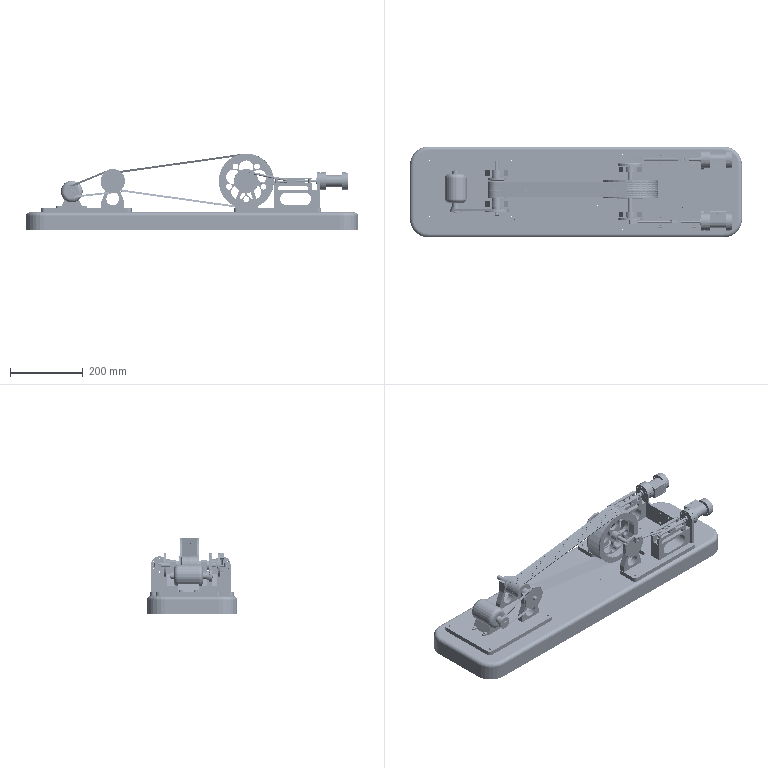Assembly | NX | mm | 63 component files | 63 solids | 1003 faces | box 915 x 250 x 212 mm | volume 14019484 mm3 | plane 402 | cylinder 384 | cone 186 | torus 16 | spline 15 | commonest cylinder face diameters 4 x86 3.3 x44 6 x42 5 x24 3 x24 12 x18 25 x18 10 x18
Bill of materials:
unnamed part 1 | 2 |  | Rectangular block with an obround (stadium-shaped) through-slot across its large side faces, four small holes on the top face near the ends, and two larger holes on one end face.
unnamed part 2 | 1 |  | Thin flat plate with rounded outer corners and a rectangular U-shaped notch with filleted inner corners cut into one edge; twelve small through-holes are spread across the plate.
unnamed part 3 | 2 |  | Rectangular flat plate with four through-holes, one near each corner.
unnamed part 4 | 4 |  | Thin circular ring (flat annulus) with a narrow rectangular-like cross-section.
unnamed part 5 | 1 |  | Single-groove V-profile pulley/sheave disc with a cylindrical hub protruding from one face and a central through-bore.
unnamed part 6 | 4 |  | Flat rectangular bar/strip with one through-hole near each end.
unnamed part 7 | 4 |  | Bridge-shaped bar with an inverted-U profile: a long top beam with a short leg at each end, filleted inner corners, and one vertical through-hole near each end on the top face.
unnamed part 8 | 2 |  | Circular disc with a central through-hole, a smaller off-center through-hole near the rim, and a shallow low boss on one face.
unnamed part 9 | 2 |  | Short solid cylinder with two rectangular circumferential grooves and a small central through-bore; one outer edge appears lightly chamfered.
unnamed part 10 | 1 |  | Thin flat plate with two raised rounded lobes at its ends; each lobe has a large central hole surrounded by six small holes, and the main body has eight medium holes in two rows. The inner corners between the lobes are filleted.
unnamed part 11 | 2 |  | Stepped cylindrical rod/shaft: a long main diameter with a short reduced-diameter section at one end.
unnamed part 12 | 1 |  | Cylindrical body with a bellows-like zigzag (convoluted) outer profile between two end flanges, plus a cylindrical hub at each end. It has a central through-bore and a small radial cross-hole in each hub.
unnamed part 13 | 1 |  | Long, slender solid cylindrical shaft or pin. Both ends step down to a short section of smaller diameter.
unnamed part 14 | 1 |  | Wheel shaped like a pulley. Its outer rim has several circumferential V-profile grooves. Inside the rim is a recessed web with five large and five small round lightening holes, around a central hub boss with a bore.
unnamed part 15 | 1 |  | Horizontal cylindrical body with rounded ends and a through-bore on its axis. It sits on a pedestal with tapered sides and a flat base. The base has four eared mounting tabs, each with a hole.
unnamed part 16 | 7 |  | Thin closed loop band with a teardrop shape. One end has a large rounded curve and the other a small rounded curve, joined by two straight tangent runs.
unnamed part 17 | 1 |  | Flat rectangular plate with rounded corners and twelve small through-holes. There is one hole near each corner. The other eight form two rectangular groups of four, each group with different spacing.
unnamed part 18 | 2 |  | Link made of a slender round rod joining two block-shaped end eyes. One block has a larger hole and chamfered corners. The other block has a rounded end and a smaller hole.
unnamed part 19 | 2 |  | Rectangular block with a rectangular notch cut in from one side, giving a U/C shape in plan. Round cross-holes pass through the side faces. A narrow rib or tongue projects from the bottom face.
unnamed part 20 | 1 |  | Stepped round shaft. One end has a collar and a short pilot spigot. The other end has stepped shoulders, a V-grooved sheave-like flange and a small end spigot.
unnamed part 21 | 2 |  | Housing with a rectangular box-shaped centre between two round end flanges. A large bore runs through along the axis. Each flange has six bolt holes in a circle. The box faces carry small holes and a set of short slots.
unnamed part 22 | 2 |  | Circular flange disc with a central bore and six bolt holes in a circle. A cylindrical hub projects from one face and a short raised face sits on the other.
unnamed part 23 | 8 |  | Plain cylindrical tube or bushing with a concentric through-bore and flat ends.
unnamed part 24 | 2 |  | Solid circular disc (blind-flange style) with six bolt holes in a circle and no central bore. A shallow raised face sits on one side and the edge is slightly chamfered.
unnamed part 25 | 4 |  | Flat plate of constant thickness with a bracket-like outline: a short semicircular lobe on top, a rectangular upper section, sides that flare outward lower down, and a rectangular base. It has a small round through-hole near the top and a large pear-shaped through-cutout below it, narrow at the top and wide and round at the bottom.
unnamed part 26 | 1 |  | Thin, long rectangular slab or pad with rounded corners in plan view and rounded or filleted edges around the top face. The bottom edge looks sharp.
unnamed part 27 | 1 |  | Long solid cylindrical rod with flat ends and two pairs of small cylindrical pins sticking out sideways. The pairs sit at two places along the rod, and in each pair the pins point in opposite directions.
unnamed part 28 | 1 |  | Thin closed-loop band with a uniform cross-section, shaped like a teardrop: a large rounded end and a small rounded end joined by two straight, converging sides. It is open in the middle and has no web.
Mates:
1. fix | base 1 component
2. concentric | base 1 arc | base_plate_1 1 edge
3. parallel | base_plate_1 1 face | base 1 face
4. concentric | support_block 2 edge | base_plate_1 1 edge
5. parallel | support_block 2 face | base_plate_1 1 face
6. parallel | support_block 1 face | support_block 2 face
7. concentric | support_block 1 edge | leg 4 edge
8. parallel | leg 4 face | support_block 1 face
9. concentric | support_block 1 edge | leg 3 edge
10. parallel | leg 3 face | support_block 1 face
11. concentric | support_block 2 edge | leg 2 edge
12. parallel | leg 2 face | support_block 2 face
13. concentric | support_block 2 edge | leg 1 edge
14. parallel | leg 1 face | support_block 2 face
15. concentric | fixed_post 8 arc | leg 4 edge
16. concentric | fixed_post 7 arc | leg 4 edge
17. concentric | fixed_post 6 arc | leg 3 edge
18. concentric | fixed_post 5 arc | leg 3 edge
19. concentric | fixed_post 8 edge | guide_plate 4 arc
20. parallel | guide_plate 4 face | leg 4 face
21. concentric | fixed_post 6 edge | guide_plate 3 arc
22. parallel | guide_plate 3 face | support_block 1 face
23. concentric | fixed_post 4 arc | leg 2 edge
24. concentric | fixed_post 3 arc | leg 2 edge
25. concentric | fixed_post 2 arc | leg 1 edge
26. concentric | fixed_post 1 arc | leg 1 edge
27. concentric | fixed_post 4 edge | guide_plate 2 arc
28. parallel | guide_plate 2 face | leg 2 face
29. concentric | fixed_post 2 edge | guide_plate 1 arc
30. parallel | guide_plate 1 face | leg 1 face
31. concentric | support_block 2 edge | piston_cylinder_mount_plate 1 arc
32. parallel | piston_cylinder_mount_plate 1 face | base 1 face
33. concentric | bracket 4 edge | base_plate_1 1 edge
34. parallel | bracket 4 face | base_plate_1 1 face
35. concentric | base_plate_1 1 edge | bracket 3 edge
36. parallel | bracket 3 face | base_plate_1 1 face
37. concentric | end_cap_2 2 edge | piston_cylinder_mount_plate 1 edge
38. concentric | end_cap_2 2 edge | piston_cylinder_mount_plate 1 edge
39. concentric | end_cap_2 1 edge | piston_cylinder_mount_plate 1 edge
40. concentric | end_cap_2 1 edge | piston_cylinder_mount_plate 1 edge
41. concentric | piston_cylinder 2 edge | end_cap_2 2 edge
42. parallel | piston_cylinder 2 face | piston_cylinder_mount_plate 1 face
43. concentric | end_cap_2 1 edge | piston_cylinder 1 edge
44. parallel | piston_cylinder 1 face | base 1 face
45. concentric | piston_cylinder 1 edge | end_cap_1 2 edge
46. concentric | end_cap_1 2 edge | piston_cylinder 1 edge
47. concentric | piston_cylinder 2 edge | end_cap_1 1 edge
48. concentric | end_cap_1 1 edge | piston_cylinder 2 edge
49. concentric | base_plate_2 1 arc | base 1 edge
50. parallel | base_plate_2 1 face | base 1 face
51. concentric | base_plate_2 1 edge | bracket 2 edge
52. parallel | bracket 2 face | base_plate_2 1 face
53. concentric | bracket 1 edge | base_plate_2 1 edge
54. parallel | bracket 1 face | bracket 2 face
55. concentric | base_plate_2 1 edge | motor 1 edge
56. parallel | motor 1 face | base 1 face
57. touch align | large_pulley_shaft 1 face | bracket 4 face
58. center | large_pulley_shaft 1 face | large_pulley_shaft 1 face | bracket 3 face | bracket 4 face
59. touch align | large_pulley 1 face | large_pulley_shaft 1 face
60. touch align | small_pulley_shaft 1 face | bracket 1 face
61. center | small_pulley_shaft 1 face | small_pulley_shaft 1 face | bracket 1 face | bracket 2 face
62. touch align | small_pulley 1 face | small_pulley_shaft 1 face
63. touch align | small_pulley 1 face | small_pulley_shaft 1 face
64. bond | bracket 2 component | assembly component
65. bond | large_belt 7 component | assembly component
66. bond | large_belt 6 component | assembly component
67. bond | large_belt 5 component | assembly component
68. bond | large_belt 4 component | assembly component
69. bond | large_belt 3 component | assembly component
70. bond | large_belt 2 component | assembly component
71. linear | assembly datumaxis | assembly cartesiancoordinatesystem | assembly cartesiancoordinatesystem | assembly cartesiancoordinatesystem | assembly cartesiancoordinatesystem | assembly cartesiancoordinatesystem | assembly cartesiancoordinatesystem | assembly cartesiancoordinatesystem
72. bond | large_belt 1 component | assembly component
73. concentric | cam 2 edge | large_pulley_shaft 1 edge
74. perpendicular | cam 2 face | large_pulley_shaft 1 face
75. perpendicular | cam 1 face | large_pulley_shaft 1 face
76. concentric | cam 1 arc | large_pulley_shaft 1 edge
77. concentric | piston_ring 4 edge | piston 2 edge
78. concentric | piston_ring 3 edge | piston 2 edge
79. concentric | piston_rod 2 edge | piston 2 edge
80. touch align | slider 2 face | piston_rod 2 face
81. distance | slider 2 face | piston 2 face
82. touch align | piston_rod 2 face | end_cap_2 2 face
83. parallel | slider 2 face | guide_plate 1 face
84. touch align | connecting_rod_1 2 face | slider 2 face
85. concentric | connecting_rod_1 2 edge | cam 1 edge
86. concentric | piston_ring 2 edge | piston 1 edge
87. concentric | piston_ring 1 edge | piston 1 edge
88. concentric | piston_rod 1 edge | piston 1 edge
89. touch align | piston_rod 1 face | end_cap_2 1 face
90. concentric | support_block 1 edge | piston_cylinder_mount_plate 1 edge
91. concentric | slider 1 edge | piston_rod 1 edge
92. parallel | slider 1 face | guide_plate 4 face
93. touch align | connecting_rod_1 1 face | slider 1 face
94. center | connecting_rod_1 1 face | connecting_rod_1 1 face | slider 1 face | slider 1 face
95. touch align | cam 2 face | connecting_rod_1 1 face
96. concentric | end_cap 2 arc | piston_cylinder 1 edge
97. parallel | piston_cylinder 1 face | end_cap 2 face
98. concentric | end_cap 1 arc | piston_cylinder 2 edge
99. parallel | end_cap 1 face | piston_cylinder 2 face
100. touch align | pulley_2 1 face | small_pulley_shaft 1 face
101. concentric | motor_shaft 1 edge | motor 1 edge
102. center | motor_shaft 1 face | motor_shaft 1 face | pulley_2 1 face | pulley_2 1 face
103. bond | belt_2 1 component | pulley_2 1 component